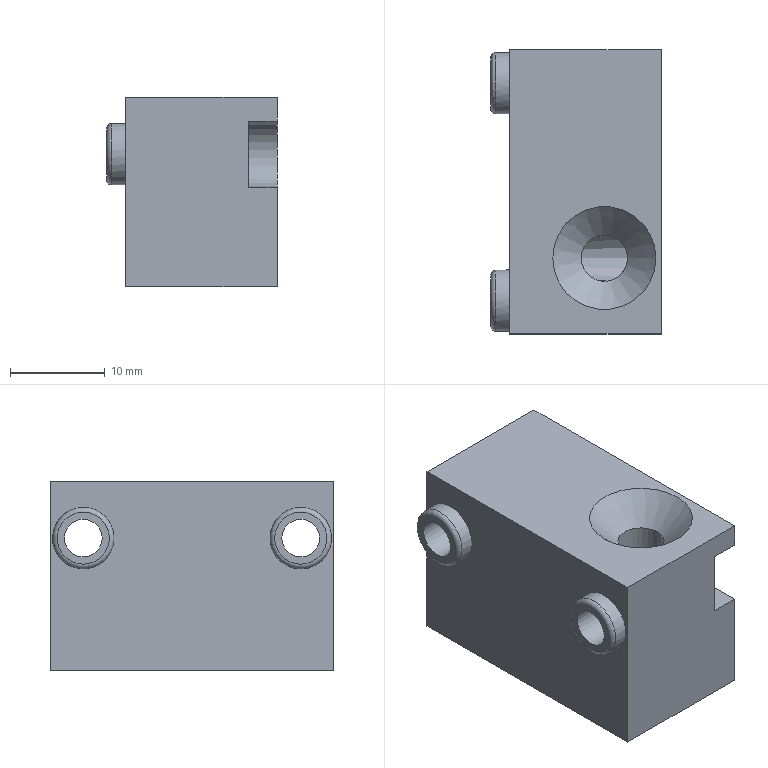Component | NX | AIR_CONN_BLOCK | 1 solid | 28 faces | volume 8569 mm3 | plane 17 | cylinder 7 | torus 2 | cone 2 | commonest cylinder face diameters 7 x2 4 x2 6.5 x2 4.9 x1